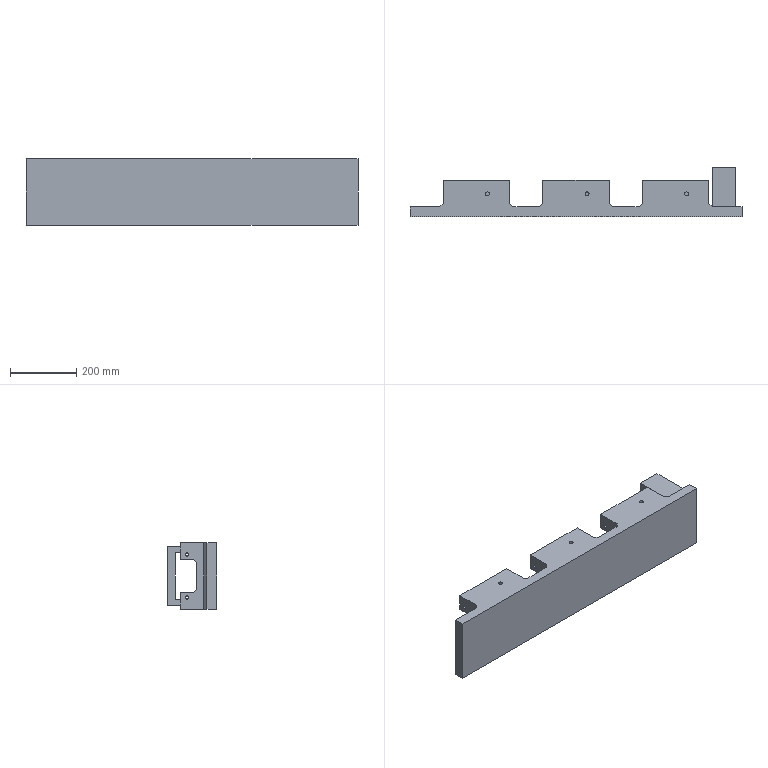Component | SolidWorks | ProductionLineBase-1 | 1 solid | 71 faces | box 1000 x 150 x 200 mm | volume 13191145 mm3 | plane 53 | cylinder 18 | commonest cylinder face diameters 10 x12 12 x6
build123d program:
from build123d import *

# Parameters (mm, degrees)
SKETCH1_2_W                     = 1000
SKETCH1_2_H                     = 200
BOSS_EXTRUDE1_DEPTH             = 30
BOSS_EXTRUDE2_REACH             = 512.784
SKETCH2_W                       = 200
SKETCH2_H                       = 80
BOSS_EXTRUDE2_DIRECTION_2_REACH = 512.784
CHAMFER1_SIZE                   = 10
CUT_EXTRUDE1_2_DEPTH            = 913.195
CUT_EXTRUDE1_2_DEPTH_BACK       = 913.195
SKETCH3_W                       = 100
SKETCH3_H                       = 100
CHAMFER2_SIZE                   = 10
CUT_EXTRUDE2_DEPTH              = 716.612
CUT_EXTRUDE2_DEPTH_BACK         = 716.612
SKETCH4_R                       = 5
SKETCH5_W                       = 70
SKETCH5_H                       = 20
BOSS_EXTRUDE3_DEPTH             = 120
BOSS_EXTRUDE4_REACH             = 550.999
SKETCH6_W                       = 70
SKETCH6_H                       = 25
SKETCH1_R                       = 6
CUT_EXTRUDE1_DEPTH              = 46


with BuildPart() as part:
    # Sketch1_2 → Boss-Extrude1 (new body)
    with BuildSketch(Plane.XY):
        Rectangle(SKETCH1_2_W, SKETCH1_2_H)
    extrude(amount=BOSS_EXTRUDE1_DEPTH)

    # Boss-Extrude2: up to this face of the body (flat: up to its plane)
    boss_extrude2_end = Plane(part.part.faces().sort_by_distance((0, 100, 15))[0])
    # Sketch2 → Boss-Extrude2 (add, up to the picked face)
    with BuildSketch(Plane(origin=(0, 0, 0), x_dir=(1, 0, 0), z_dir=(0, 1, 0)), mode=Mode.PRIVATE) as boss_extrude2_sk1:
        with Locations((-300, -70)):
            Rectangle(SKETCH2_W, SKETCH2_H)
    boss_extrude2_tool1 = split(extrude(boss_extrude2_sk1.sketch, amount=BOSS_EXTRUDE2_REACH, mode=Mode.PRIVATE), bisect_by=boss_extrude2_end, keep=Keep.BOTH, mode=Mode.PRIVATE)
    # Sketch2 → Boss-Extrude2 (add, up to the picked face)
    with BuildSketch(Plane(origin=(0, 0, 0), x_dir=(1, 0, 0), z_dir=(0, 1, 0)), mode=Mode.PRIVATE) as boss_extrude2_sk2:
        with Locations((0, -70)):
            Rectangle(SKETCH2_W, SKETCH2_H)
    boss_extrude2_tool2 = split(extrude(boss_extrude2_sk2.sketch, amount=BOSS_EXTRUDE2_REACH, mode=Mode.PRIVATE), bisect_by=boss_extrude2_end, keep=Keep.BOTH, mode=Mode.PRIVATE)
    # Sketch2 → Boss-Extrude2 (add, up to the picked face)
    with BuildSketch(Plane(origin=(0, 0, 0), x_dir=(1, 0, 0), z_dir=(0, 1, 0)), mode=Mode.PRIVATE) as boss_extrude2_sk3:
        with Locations((300, -70)):
            Rectangle(SKETCH2_W, SKETCH2_H)
    boss_extrude2_tool3 = split(extrude(boss_extrude2_sk3.sketch, amount=BOSS_EXTRUDE2_REACH, mode=Mode.PRIVATE), bisect_by=boss_extrude2_end, keep=Keep.BOTH, mode=Mode.PRIVATE)
    add(boss_extrude2_tool1.solids().sort_by(Axis((-300, 0, 70), (0, 1, 0)))[0])
    add(boss_extrude2_tool2.solids().sort_by(Axis((0, 0, 70), (0, 1, 0)))[0])
    add(boss_extrude2_tool3.solids().sort_by(Axis((300, 0, 70), (0, 1, 0)))[0])

    # Boss-Extrude2 direction 2: up to this face of the body (flat: up to its plane)
    boss_extrude2_direction_2_end = Plane(part.part.faces().sort_by_distance((0, -100, 15))[0])
    # Sketch2 → Boss-Extrude2 direction 2 (add, up to the picked face)
    with BuildSketch(Plane(origin=(0, 0, 0), x_dir=(1, 0, 0), z_dir=(0, 1, 0)), mode=Mode.PRIVATE) as boss_extrude2_direction_2_sk1:
        with Locations((-300, -70)):
            Rectangle(SKETCH2_W, SKETCH2_H)
    boss_extrude2_direction_2_tool1 = split(extrude(boss_extrude2_direction_2_sk1.sketch, amount=-BOSS_EXTRUDE2_DIRECTION_2_REACH, mode=Mode.PRIVATE), bisect_by=boss_extrude2_direction_2_end, keep=Keep.BOTH, mode=Mode.PRIVATE)
    # Sketch2 → Boss-Extrude2 direction 2 (add, up to the picked face)
    with BuildSketch(Plane(origin=(0, 0, 0), x_dir=(1, 0, 0), z_dir=(0, 1, 0)), mode=Mode.PRIVATE) as boss_extrude2_direction_2_sk2:
        with Locations((0, -70)):
            Rectangle(SKETCH2_W, SKETCH2_H)
    boss_extrude2_direction_2_tool2 = split(extrude(boss_extrude2_direction_2_sk2.sketch, amount=-BOSS_EXTRUDE2_DIRECTION_2_REACH, mode=Mode.PRIVATE), bisect_by=boss_extrude2_direction_2_end, keep=Keep.BOTH, mode=Mode.PRIVATE)
    # Sketch2 → Boss-Extrude2 direction 2 (add, up to the picked face)
    with BuildSketch(Plane(origin=(0, 0, 0), x_dir=(1, 0, 0), z_dir=(0, 1, 0)), mode=Mode.PRIVATE) as boss_extrude2_direction_2_sk3:
        with Locations((300, -70)):
            Rectangle(SKETCH2_W, SKETCH2_H)
    boss_extrude2_direction_2_tool3 = split(extrude(boss_extrude2_direction_2_sk3.sketch, amount=-BOSS_EXTRUDE2_DIRECTION_2_REACH, mode=Mode.PRIVATE), bisect_by=boss_extrude2_direction_2_end, keep=Keep.BOTH, mode=Mode.PRIVATE)
    add(boss_extrude2_direction_2_tool1.solids().sort_by(Axis((-300, 0, 70), (0, -1, 0)))[0])
    add(boss_extrude2_direction_2_tool2.solids().sort_by(Axis((0, 0, 70), (0, -1, 0)))[0])
    add(boss_extrude2_direction_2_tool3.solids().sort_by(Axis((300, 0, 70), (0, -1, 0)))[0])

    # Chamfer1
    chamfer1_edges = [part.edges().sort_by_distance(p)[0] for p in [
        (-200, 0, 30),
        (-400, 0, 30),
        (100, 0, 30),
        (-100, 0, 30),
        (400, 0, 30),
        (200, 0, 30),
    ]]
    chamfer(chamfer1_edges, length=CHAMFER1_SIZE)

    # Sketch3 → Cut-Extrude1_2 (cut, two sides: drawn at the far end of the back side and taken through both)
    with BuildSketch(Plane.ZY.offset(400).offset(-CUT_EXTRUDE1_2_DEPTH_BACK)):
        with Locations((110, 0)):
            Rectangle(SKETCH3_W, SKETCH3_H)
    extrude(amount=CUT_EXTRUDE1_2_DEPTH + CUT_EXTRUDE1_2_DEPTH_BACK, mode=Mode.SUBTRACT)

    # Chamfer2
    chamfer2_edges = [part.edges().sort_by_distance(p)[0] for p in [
        (-300, -50, 60),
        (0, -50, 60),
        (300, -50, 60),
        (-300, 50, 60),
        (0, 50, 60),
        (300, 50, 60),
    ]]
    chamfer(chamfer2_edges, length=CHAMFER2_SIZE)

    # Sketch4 → Cut-Extrude2 (cut, two sides: drawn at the far end of the back side and taken through both)
    with BuildSketch(Plane(origin=(-200, 0, 0), x_dir=(0, 0, -1), z_dir=(1, 0, 0)).offset(-CUT_EXTRUDE2_DEPTH_BACK)):
        with Locations((-90, -65)):
            Circle(SKETCH4_R)
        with Locations((-90, 65)):
            Circle(SKETCH4_R)
    extrude(amount=CUT_EXTRUDE2_DEPTH + CUT_EXTRUDE2_DEPTH_BACK, mode=Mode.SUBTRACT)

    # Sketch5 → Boss-Extrude3 (add)
    with BuildSketch(Plane.XY.offset(30)):
        with Locations((445, 80)):
            Rectangle(SKETCH5_W, SKETCH5_H)
        with Locations((445, -80)):
            Rectangle(SKETCH5_W, SKETCH5_H)
    extrude(amount=BOSS_EXTRUDE3_DEPTH)

    # Sketch6 → Boss-Extrude4 (add, up to next)
    with BuildSketch(Plane.XZ.offset(-70), mode=Mode.PRIVATE) as boss_extrude4_sk1:
        with Locations((445, 137.5)):
            Rectangle(SKETCH6_W, SKETCH6_H)
    boss_extrude4_tool1 = extrude(boss_extrude4_sk1.sketch, amount=BOSS_EXTRUDE4_REACH, mode=Mode.PRIVATE) - part.part
    add(boss_extrude4_tool1.solids().sort_by_distance((445, 70, 137.5))[0])

    # Sketch1 → Cut-Extrude1 (cut)
    with BuildSketch(Plane.XZ.offset(100)):
        with Locations((33.291, 69.045)):
            Circle(SKETCH1_R)
        with Locations((333.291, 69.045)):
            Circle(SKETCH1_R)
        with Locations((-266.709, 69.045)):
            Circle(SKETCH1_R)
    extrude(amount=-CUT_EXTRUDE1_DEPTH, mode=Mode.SUBTRACT)


solid = part.part

# Placed as in the assembly
solid = solid.moved(Location((0, 0, 0), (-90, 0, 0)))